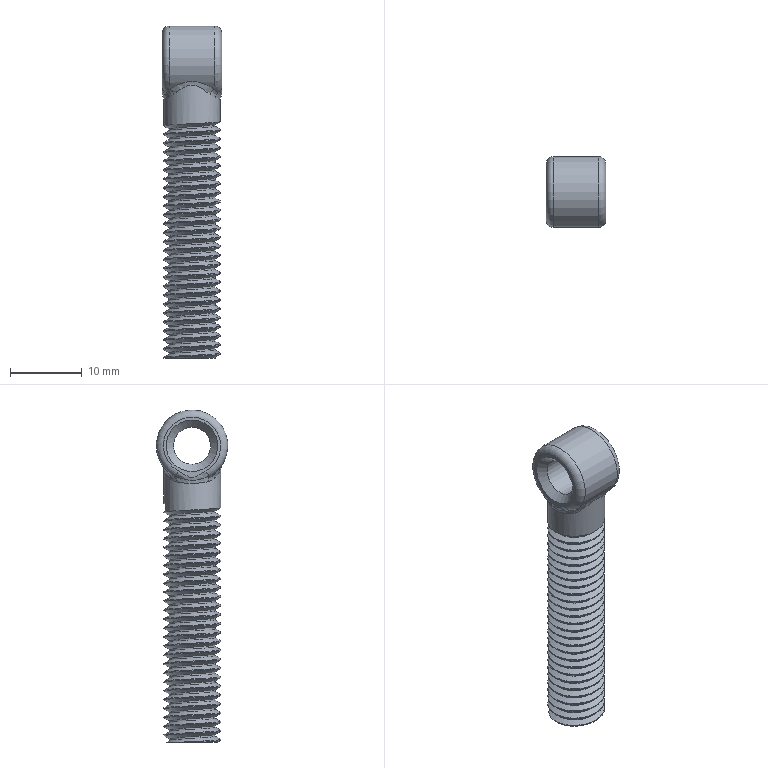Component | NX | BOLT | 1 solid | 50 faces | volume 1933 mm3 | cylinder 30 | spline 12 | plane 4 | cone 2 | torus 2 | commonest cylinder face diameters 7.94 x27 10 x1 5.2 x1 6.466 x1